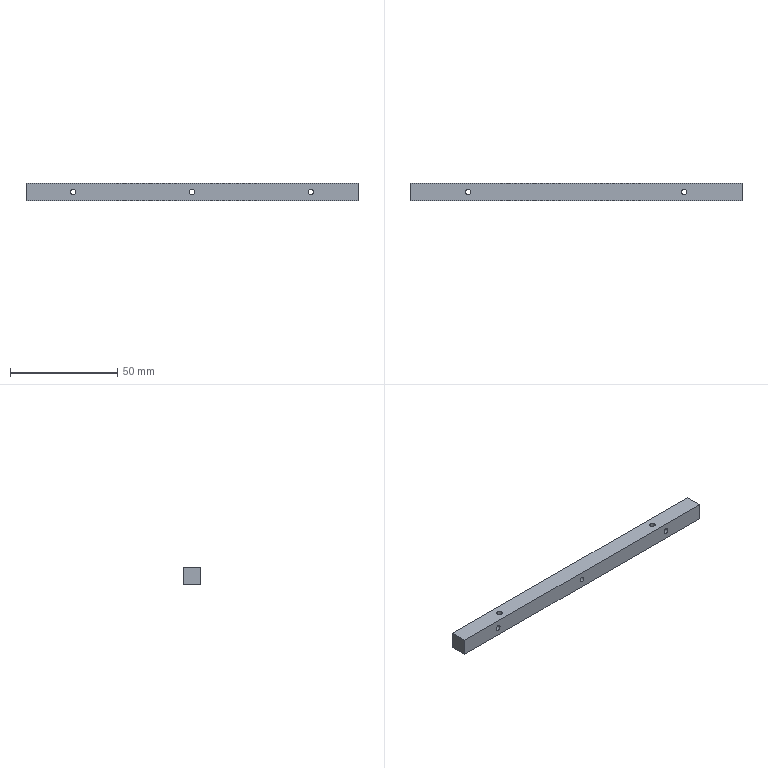CAM job | Mastercam | mm | 8 operations | part box 154.55 x 8 x 8
1. Facing | 24 - 100 平铣刀
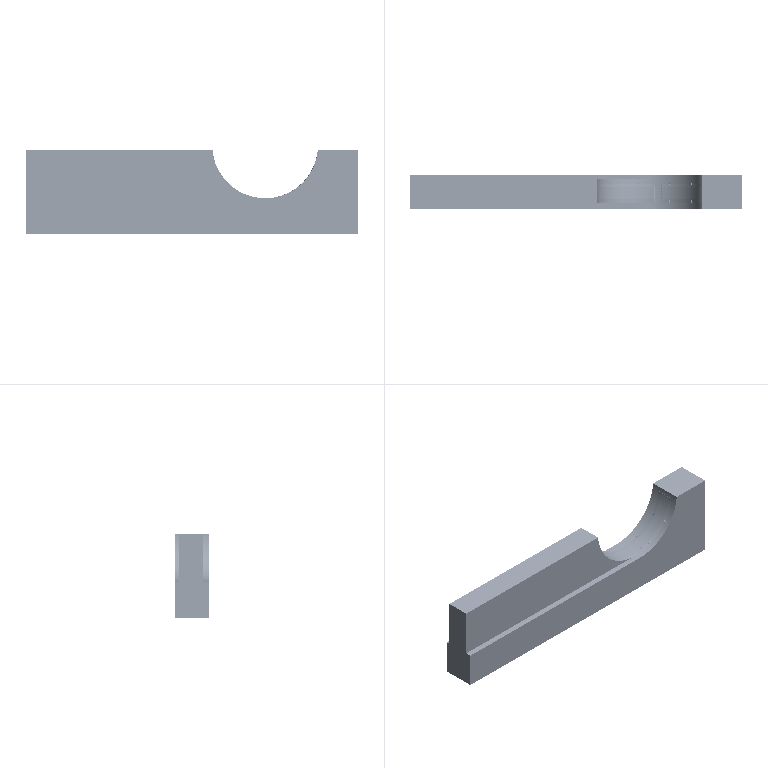2. Contour (Ramp) | 10 - 10 平铣刀
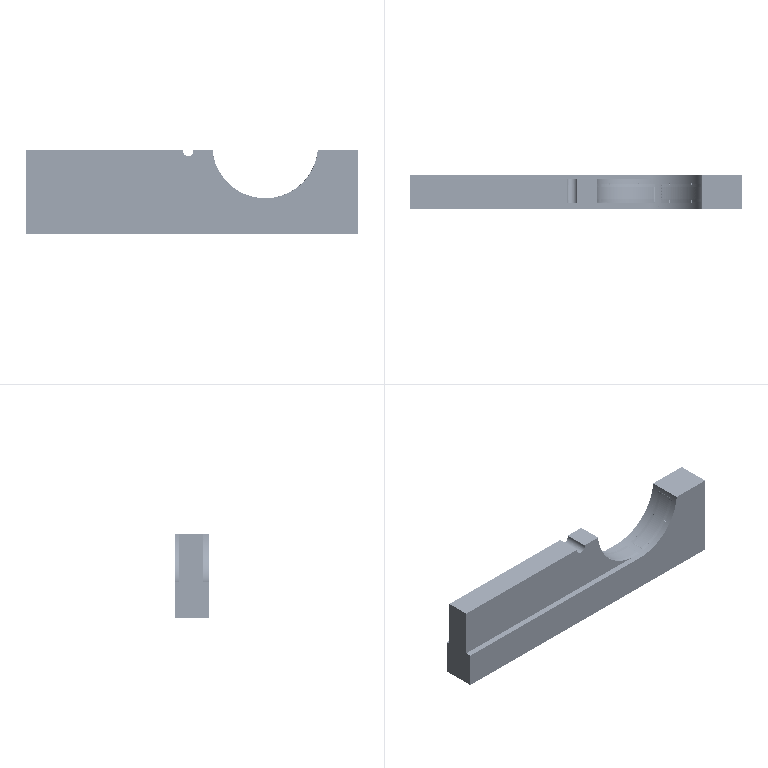3. Contour (2D) | 10 - 10 平铣刀
4. Drill/Counterbore | 7 - 4 倒角刀
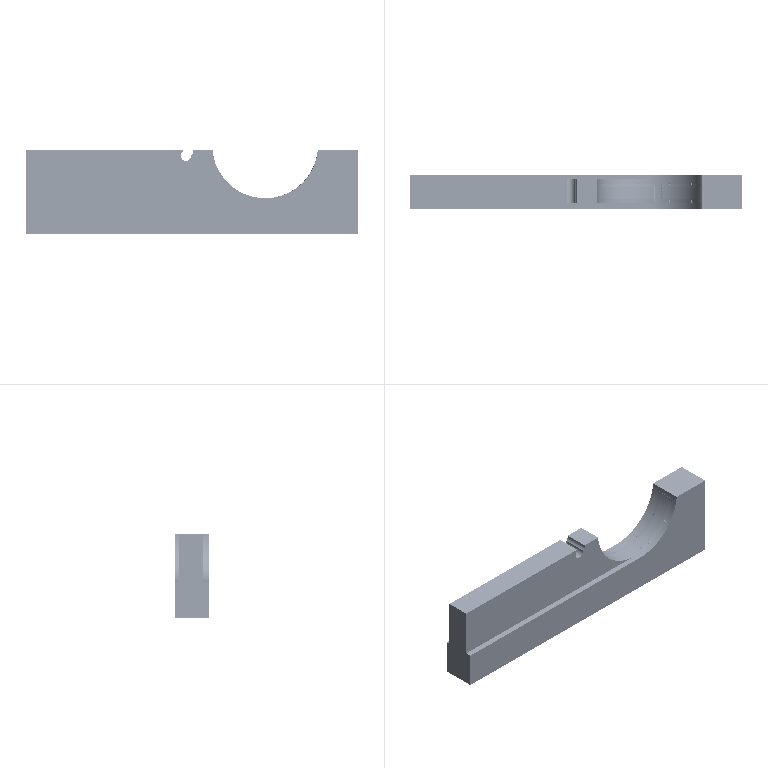5. Contour (2D chamfer) | 7 - 4 倒角刀
6. Facing | 24 - 100 平铣刀
7. Contour (2D chamfer) | 7 - 4 倒角刀
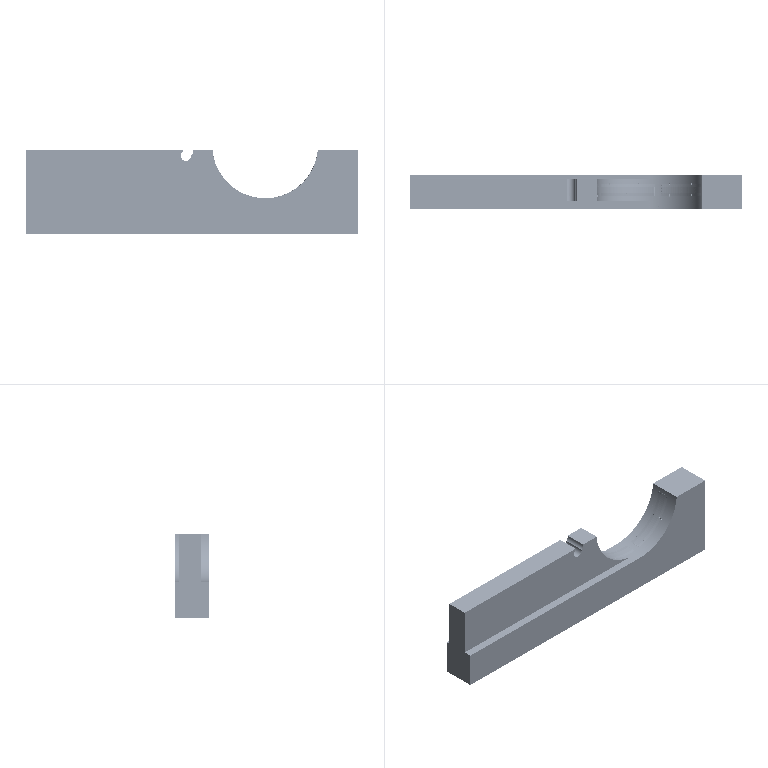8. Drill/Counterbore | 7 - 4 倒角刀